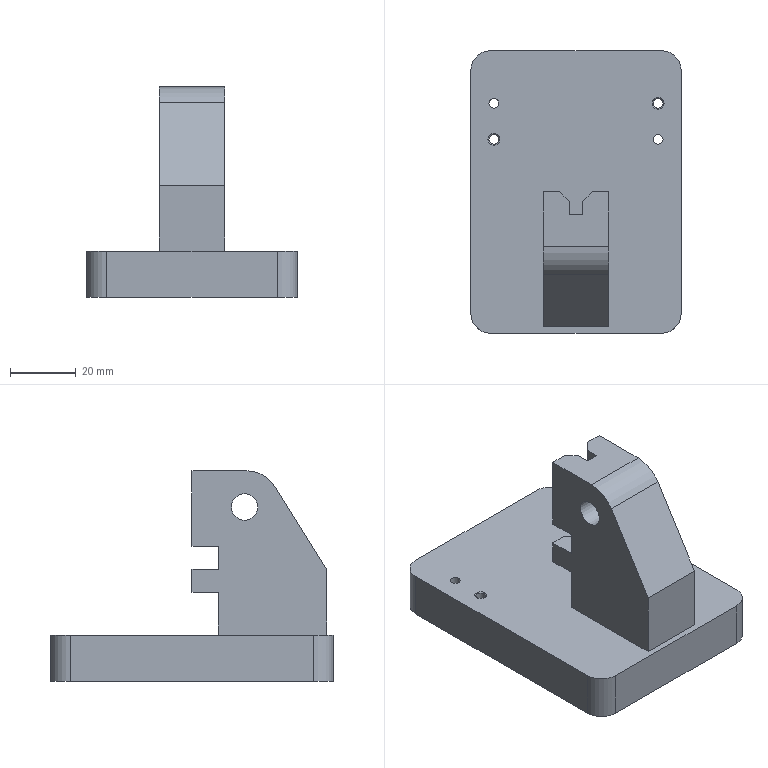Component | NX | BASE | 1 solid | 42 faces | volume 106191 mm3 | plane 30 | cylinder 10 | cone 2 | commonest cylinder face diameters 12 x4 3 x4 20 x1 8 x1